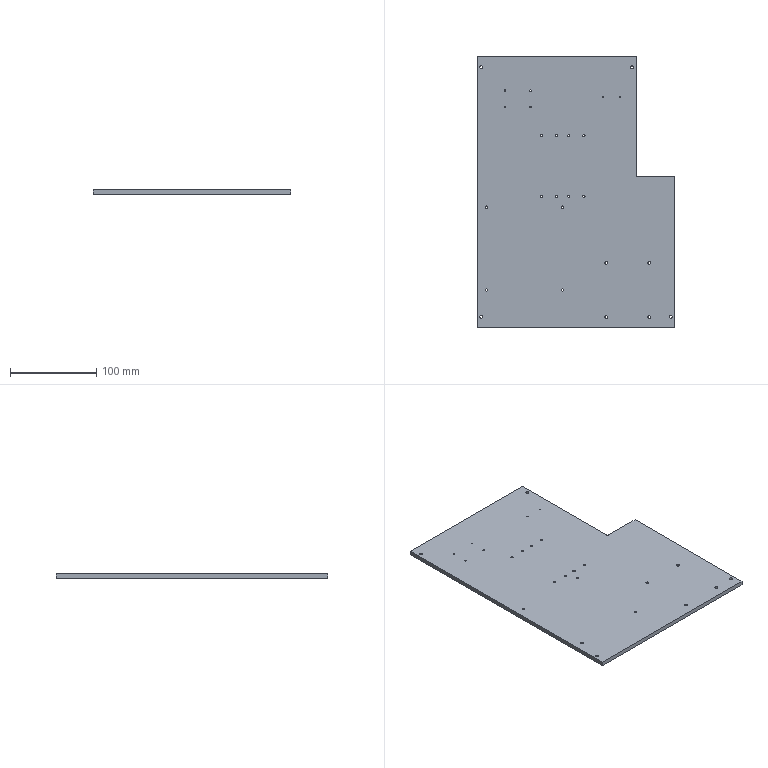CAM job | Mastercam | mm | 6 operations | part box 230 x 315.9 x 5
1. Contour (Ramp) | 9 - 10 平铣刀
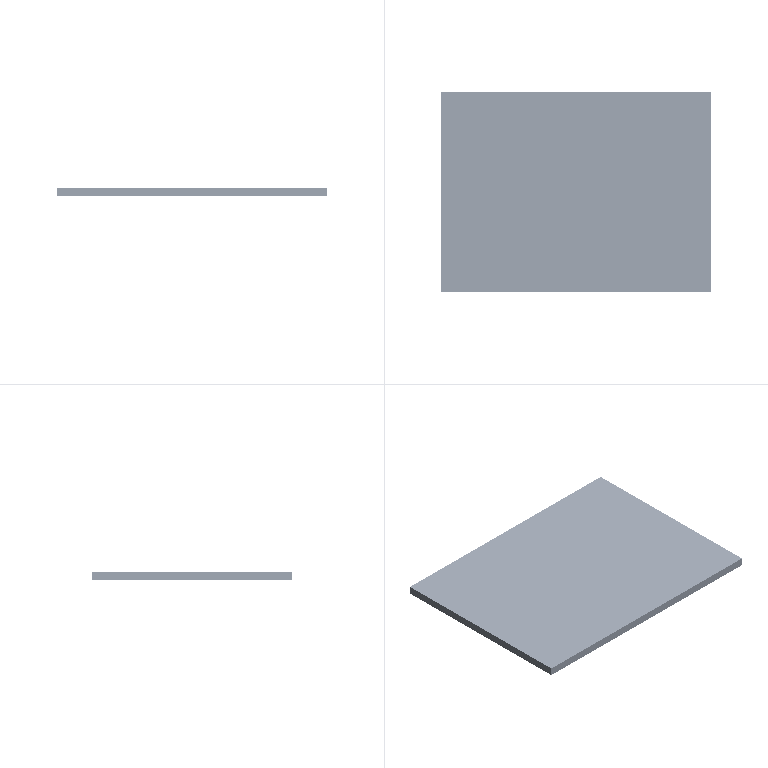2. Contour (2D) | 10 - 10 平铣刀
3. Contour (2D) | 3 - 3 平铣刀
4. Contour (2D) | 2 - 2 平铣刀
5. Drill/Counterbore | 7 - 4 倒角刀
6. Contour (2D chamfer) | 7 - 4 倒角刀